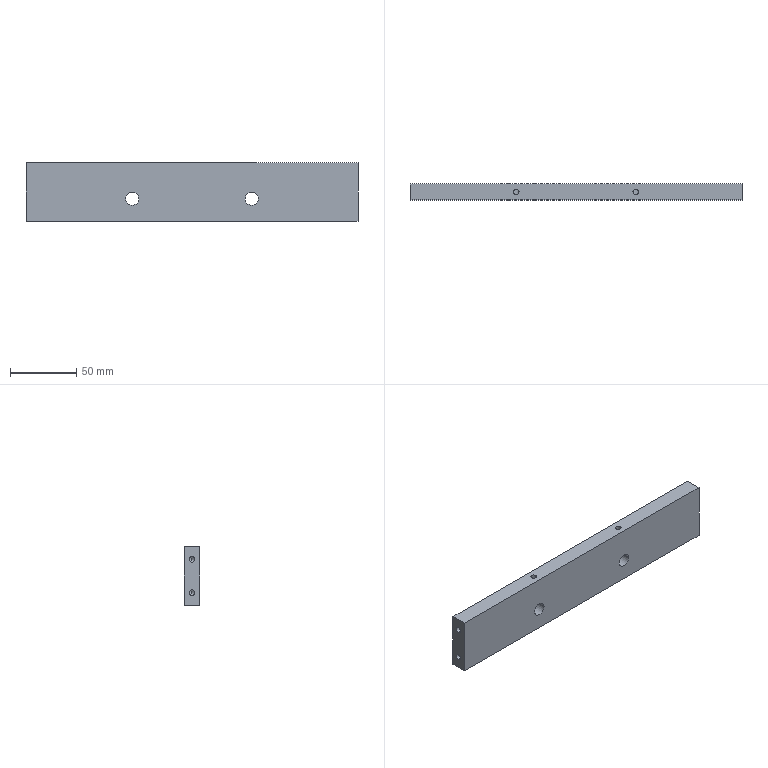Component | SolidWorks | STB-08-043-1 | 1 solid | 42 faces | box 250 x 12 x 44 mm | volume 128161 mm3 | cylinder 22 | cone 14 | plane 6 | commonest cylinder face diameters 4.2 x12 3.3 x6 10 x4 | material 6061 Alloy
build123d program:
from build123d import *

# Parameters (mm, degrees)
SKETCH1_W                  = 44
SKETCH1_H                  = 250
EXTRUDE1_DEPTH             = 6
M5_TAPPED_HOLE1_AT_2_COUNT = 2
M5_TAPPED_HOLE1_AT_2_PITCH = 25
M4_TAPPED_HOLE1_D          = 3.3
M4_TAPPED_HOLE1_DEPTH      = 10
M4_TAPPED_HOLE1_TIP        = 0.9914
CUT_EXTRUDE1_REACH         = 129.487
SKETCH6_R                  = 5
M5_TAPPED_HOLE2_REACH      = 134.654
M5_TAPPED_HOLE2_BORE_R     = 2.1


with BuildPart() as part:
    # Sketch1 → Extrude1 (new, symmetric)
    with BuildSketch(Plane(origin=(0, 0, 0), x_dir=(1, 0, 0), z_dir=(0, 1, 0))):
        Rectangle(SKETCH1_W, SKETCH1_H)
    extrude(amount=EXTRUDE1_DEPTH, both=True)

    # Sketch2 → M5 Tapped Hole1 (revolve, cut)
    with BuildSketch(Plane(origin=(-12.5, 0, 125), x_dir=(0, -1, 0), z_dir=(1, 0, 0))):
        Polygon((0, 0), (0, 20.262), (2.1, 19), (2.1, 0), align=None)
    m5_tapped_hole1 = revolve(axis=Axis((-12.5, 0, 131.35), (0, 0, -1)), mode=Mode.SUBTRACT)

    # M5 Tapped Hole1 at 2: M5 Tapped Hole1 ×2
    with Locations(*[(i * M5_TAPPED_HOLE1_AT_2_PITCH, 0, 0) for i in range(1, M5_TAPPED_HOLE1_AT_2_COUNT)]):
        add(m5_tapped_hole1, mode=Mode.SUBTRACT)

    # Mirror1: M5 Tapped Hole1 across plane
    add(m5_tapped_hole1.mirror(Plane.XY), mode=Mode.SUBTRACT)

    # Mirror1 copy 1 sketch → Mirror1 copy 1 (revolve, cut)
    with BuildSketch(Plane(origin=(12.5, 0, -125), x_dir=(0, -1, 0), z_dir=(1, 0, 0))):
        Polygon((0, 0), (0, -20.262), (2.1, -19), (2.1, 0), align=None)
    revolve(axis=Axis((12.5, 0, -131.35), (0, 0, -1)), mode=Mode.SUBTRACT)

    # M4 Tapped Hole1
    with Locations(Plane.ZY.offset(22)):
        with Locations((90, 0), (0, 0), (-90, 0)):
            Hole(M4_TAPPED_HOLE1_D / 2, depth=M4_TAPPED_HOLE1_DEPTH)
            with Locations((0, 0, -(M4_TAPPED_HOLE1_DEPTH + M4_TAPPED_HOLE1_TIP / 2))):  # 118° drill point
                Cone(0, M4_TAPPED_HOLE1_D / 2, M4_TAPPED_HOLE1_TIP, mode=Mode.SUBTRACT)

    # Sketch6 → Cut-Extrude1 (cut, up to next)
    with BuildSketch(Plane(origin=(0, 6, 0), x_dir=(1, 0, 0), z_dir=(0, 1, 0)), mode=Mode.PRIVATE) as cut_extrude1_sk1:
        with Locations(Location((-5, -45, 0), (0, 0, 270))):
            Circle(SKETCH6_R)
    cut_extrude1_tool1 = extrude(cut_extrude1_sk1.sketch, amount=-CUT_EXTRUDE1_REACH, mode=Mode.PRIVATE) & part.part
    # Sketch6 → Cut-Extrude1 (cut, up to next)
    with BuildSketch(Plane(origin=(0, 6, 0), x_dir=(1, 0, 0), z_dir=(0, 1, 0)), mode=Mode.PRIVATE) as cut_extrude1_sk2:
        with Locations(Location((-5, 45, 0), (0, 0, 270))):
            Circle(SKETCH6_R)
    cut_extrude1_tool2 = extrude(cut_extrude1_sk2.sketch, amount=-CUT_EXTRUDE1_REACH, mode=Mode.PRIVATE) & part.part
    add(cut_extrude1_tool1.solids().sort_by_distance((-5, 6, 45))[0], mode=Mode.SUBTRACT)
    add(cut_extrude1_tool2.solids().sort_by_distance((-5, 6, -45))[0], mode=Mode.SUBTRACT)

    # M5 Tapped Hole2 bore → M5 Tapped Hole2 (cut, up to next)
    with BuildSketch(Plane(origin=(22, 0, 0), x_dir=(0, 0, -1), z_dir=(1, 0, 0)), mode=Mode.PRIVATE) as m5_tapped_hole2_sk1:
        with Locations((45, 0)):
            Circle(M5_TAPPED_HOLE2_BORE_R)
    m5_tapped_hole2_tool1 = extrude(m5_tapped_hole2_sk1.sketch, amount=-M5_TAPPED_HOLE2_REACH, mode=Mode.PRIVATE) & part.part
    # M5 Tapped Hole2 bore → M5 Tapped Hole2 (cut, up to next)
    with BuildSketch(Plane(origin=(22, 0, 0), x_dir=(0, 0, -1), z_dir=(1, 0, 0)), mode=Mode.PRIVATE) as m5_tapped_hole2_sk2:
        with Locations((-45, 0)):
            Circle(M5_TAPPED_HOLE2_BORE_R)
    m5_tapped_hole2_tool2 = extrude(m5_tapped_hole2_sk2.sketch, amount=-M5_TAPPED_HOLE2_REACH, mode=Mode.PRIVATE) & part.part
    add(m5_tapped_hole2_tool1.solids().sort_by_distance((22, 0, -45))[0], mode=Mode.SUBTRACT)
    add(m5_tapped_hole2_tool2.solids().sort_by_distance((22, 0, 45))[0], mode=Mode.SUBTRACT)


solid = part.part

# Placed as in the assembly
solid = solid.moved(Location((-104.904, 237.999, -7), (0, -90, 0)))